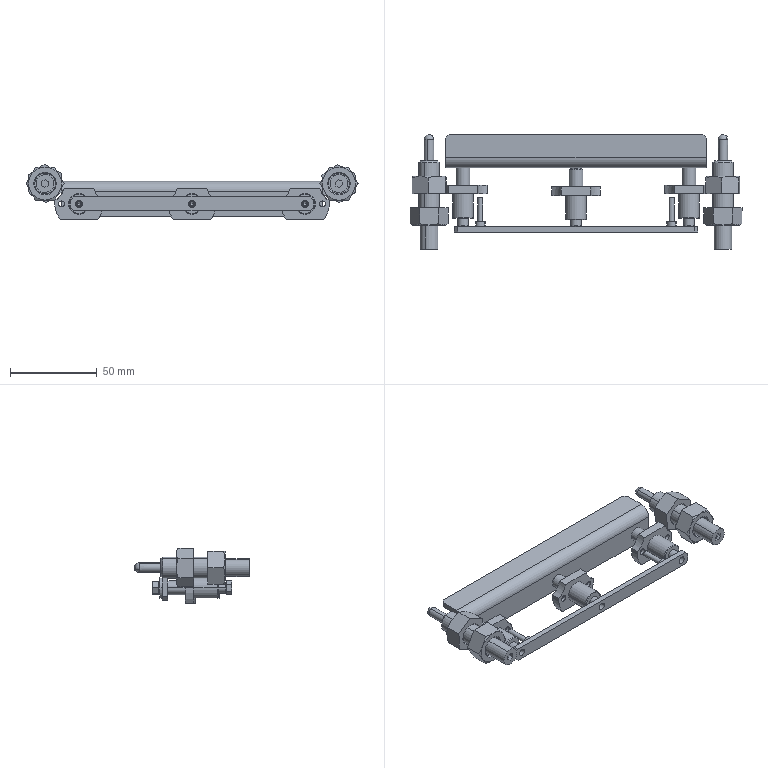Assembly | SolidWorks | mm | 28 component files | 28 solids | 468 faces | box 190.94 x 66 x 31.66 mm | volume 51082 mm3 | plane 186 | cylinder 150 | cone 116 | torus 12 | sphere 4 | commonest cylinder face diameters 6 x25 12 x25 4 x18 3.5 x12 28 x9 5.5 x8 22.6 x6 6.7 x6
Bill of materials:
LME21-d6 | 3 |  | Flanged sleeve: a cylindrical sleeve with a through bore, sticking out from one face of a flat flange plate. The flange has two through holes, one on each side of the sleeve.
MTCTV2104DJ006-000-0002PressurePlate | 1 |  | Long, thin L-shaped angle profile with a rounded bend. One leg has three round through holes along its length.
MTCTV2104DJ006-000-0004LimitStrip | 1 |  | Thin, flat rectangular bar with three round through holes along its length and chamfered corners at both ends.
SGE14-D6-L34-F8-B6-P4-N3 | 3 |  | Stepped cylindrical pin: a larger-diameter main body and a shorter, smaller-diameter spigot at one end. The larger end has a centered axial hole.
TAC01-M3-L14 | 2 |  | Shape like a socket-head screw: a cylindrical head with a hexagonal recess, and a plain cylindrical shank with a chamfered tip.
TBK51-M12 | 4 |  | Hexagonal nut-like prism with a central round through bore and a chamfered outer edge on one face.
TBK51-M4 | 3 |  | Hexagonal nut-like prism with a central round through bore, chamfered on one face, similar to the other hex part but shown in a different orientation.
TBN12-4 | 3 |  | Flat circular washer-like ring: a thin disc with a central round hole.
TBN42-4 | 3 |  | Flat split ring: an annular ring with one radial cut through it.
YWL-D8-L10 | 3 |  | Thin-walled cylindrical tube with plain square-cut ends.
ZAP07-M12-H15 | 2 |  | Stepped cylindrical shaft with three diameters: a middle section, the largest; a smaller pin at one end with a rounded tip; and a section at the other end with a hexagonal socket in its end face.
Mates:
1. coincident | LME21-d6-1 face at (-60.536, 63.25, 217.788) dir (0, 1, 0) | YWL-D8-L10-1 face at (-57.536, 63.25, 217.788) dir (0, -1, 0)
2. concentric | LME21-d6-1 face at (-57.536, 63.25, 217.788) dir (0, 1, 0) r 3 | YWL-D8-L10-1 face at (-57.536, 63.25, 217.788) dir (0, 1, 0) r 4
3. coincident | LME21-d6-2 face at (-125.536, 62.25, 217.788) dir (0, 1, 0) | YWL-D8-L10-2 face at (-122.536, 62.25, 217.788) dir (0, -1, 0)
4. concentric | LME21-d6-2 face at (-122.536, 62.25, 217.788) dir (0, 1, 0) r 3 | YWL-D8-L10-2 face at (-122.536, 72.25, 217.788) dir (0, -1, 0) r 4
5. coincident | LME21-d6-3 face at (-190.536, 63.25, 217.788) dir (0, 1, 0) | YWL-D8-L10-3 face at (-187.536, 63.25, 217.788) dir (0, -1, 0)
6. concentric | LME21-d6-3 face at (-187.536, 63.25, 217.788) dir (0, 1, 0) r 3 | YWL-D8-L10-3 face at (-187.536, 63.25, 217.788) dir (0, 1, 0) r 4
7. coincident | YWL-D8-L10-1 face at (-57.536, 73.25, 217.788) dir (0, 1, 0) | MTCTV2104DJ006-000-0002PressurePlate-1 face at (-122.536, 73.25, 220.788) dir (0, -1, 0)
8. concentric | YWL-D8-L10-1 face at (-57.536, 63.25, 217.788) dir (0, 1, 0) r 4 | MTCTV2104DJ006-000-0002PressurePlate-1 face at (-57.536, 73.25, 217.788) dir (0, -1, 0) r 2.5
9. concentric | YWL-D8-L10-3 face at (-187.536, 63.25, 217.788) dir (0, 1, 0) r 3.35 | MTCTV2104DJ006-000-0002PressurePlate-1 face at (-187.536, 73.25, 217.788) dir (0, -1, 0) r 2.5
10. coincident | MTCTV2104DJ006-000-0002PressurePlate-1 face at (-122.536, 73.25, 220.788) dir (0, -1, 0) | SGE14-D6-L34-F8-B6-P4-N3-1 face at (-57.536, 73.25, 220.588) dir (0, 1, 0)
11. concentric | LME21-d6-1 face at (-57.536, 63.25, 217.788) dir (0, 1, 0) r 3 | SGE14-D6-L34-F8-B6-P4-N3-1 face at (-57.536, 81.25, 217.788) dir (0, -1, 0) r 3
12. coincident | MTCTV2104DJ006-000-0002PressurePlate-1 face at (-122.536, 73.25, 220.788) dir (0, -1, 0) | SGE14-D6-L34-F8-B6-P4-N3-2 face at (-187.536, 73.25, 220.588) dir (0, 1, 0)
13. concentric | LME21-d6-3 face at (-187.536, 63.25, 217.788) dir (0, 1, 0) r 3 | SGE14-D6-L34-F8-B6-P4-N3-2 face at (-187.536, 81.25, 217.788) dir (0, -1, 0) r 3
14. concentric | LME21-d6-2 face at (-122.536, 62.25, 217.788) dir (0, 1, 0) r 3 | SGE14-D6-L34-F8-B6-P4-N3-3 face at (-122.536, 81.25, 217.788) dir (0, -1, 0) r 3
15. coincident | MTCTV2104DJ006-000-0002PressurePlate-1 face at (-122.536, 73.25, 220.788) dir (0, -1, 0) | SGE14-D6-L34-F8-B6-P4-N3-3 face at (-122.536, 73.25, 220.588) dir (0, 1, 0)
16. coincident | MTCTV2104DJ006-000-0002PressurePlate-1 face at (-122.536, 76.25, 220.788) dir (0, 1, 0) | TBN12-4-1 face at (-187.536, 76.25, 217.788) dir (0, -1, 0)
17. concentric | SGE14-D6-L34-F8-B6-P4-N3-2 face at (-187.536, 81.25, 217.788) dir (0, -1, 0) r 2 | TBN12-4-1 face at (-187.536, 76.25, 217.788) dir (0, 1, 0) r 2.15
18. concentric | SGE14-D6-L34-F8-B6-P4-N3-2 face at (-187.536, 81.25, 217.788) dir (0, -1, 0) r 2 | TBN42-4-1 face at (-187.536, 78.75, 217.788) dir (0, -1, 0) r 2.4
19. coincident | TBN12-4-1 face at (-187.536, 77.85, 217.788) dir (0, 1, 0) | TBN42-4-1 plane at (-187.536, 77.85, 217.788) dir (0, 1, 0)
20. concentric | SGE14-D6-L34-F8-B6-P4-N3-2 face at (-187.536, 81.25, 217.788) dir (0, -1, 0) r 2 | TBK51-M4-1 face at (-187.536, 31.95, 217.788) dir (0, 1, 0) r 2
21. coincident | SGE14-D6-L34-F8-B6-P4-N3-1 face at (-57.536, 39.25, 217.788) dir (0, -1, 0) | TAC01-M3-L14-1 face at (-67.536, 39.25, 217.788) dir (0, -1, 0)
22. coincident | SGE14-D6-L34-F8-B6-P4-N3-2 face at (-187.536, 39.25, 217.788) dir (0, -1, 0) | TAC01-M3-L14-2 face at (-177.536, 39.25, 217.788) dir (0, -1, 0)
23. coincident | ZAP07-M12-H15-1 face at (-33.529, 42.25, 233.401) dir (0, -1, 0) | ZAP07-M12-H15-2 face at (-201.616, 42.25, 232.066) dir (0, -1, 0)
24. concentric | ZAP07-M12-H15-1 face at (-38.036, -24.75, 229.44) dir (0, 1, 0) r 6 | TBK51-M12-1 face at (-38.036, 90.25, 229.44) dir (0, -1, 0) r 6
25. concentric | ZAP07-M12-H15-2 face at (-207.036, -24.75, 229.492) dir (0, 1, 0) r 6 | TBK51-M12-2 face at (-207.036, 90.25, 229.492) dir (0, -1, 0) r 6
26. concentric | ZAP07-M12-H15-2 face at (-207.036, -24.75, 229.492) dir (0, 1, 0) r 6 | TBK51-M12-3 face at (-207.036, 18.25, 229.492) dir (0, 1, 0) r 6
27. concentric | ZAP07-M12-H15-1 face at (-38.036, -24.75, 229.44) dir (0, 1, 0) r 6 | TBK51-M12-4 face at (-38.036, 18.25, 229.44) dir (0, 1, 0) r 6
28. coincident | SGE14-D6-L34-F8-B6-P4-N3-3 face at (-122.536, 39.25, 217.788) dir (0, -1, 0) | MTCTV2104DJ006-000-0004LimitStrip-1 face at (-122.536, 39.25, 217.788) dir (0, 1, 0)
29. concentric | SGE14-D6-L34-F8-B6-P4-N3-2 face at (-187.536, 81.25, 217.788) dir (0, -1, 0) r 3 | MTCTV2104DJ006-000-0004LimitStrip-1 face at (-187.536, 39.25, 217.788) dir (0, 1, 0) r 2
30. concentric | SGE14-D6-L34-F8-B6-P4-N3-1 face at (-57.536, 81.25, 217.788) dir (0, -1, 0) r 3 | MTCTV2104DJ006-000-0004LimitStrip-1 face at (-57.536, 39.25, 217.788) dir (0, 1, 0) r 2
31. coincident | TBK51-M4-1 face at (-189.834, 78.75, 217.882) dir (0, -1, 0) | TBN42-4-1 face at (-189.252, 78.75, 216.667) dir (0, 1, 0)